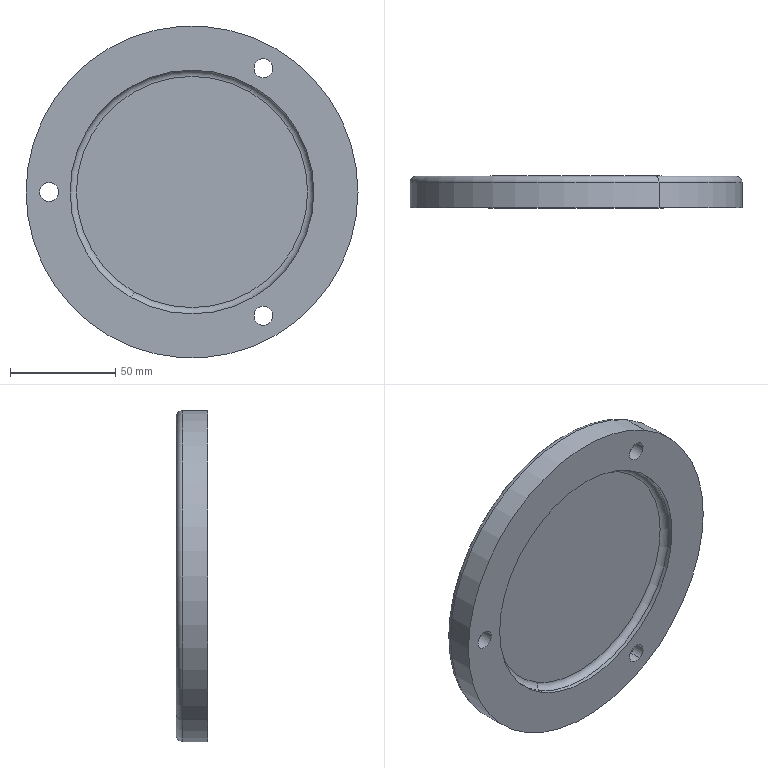Component | SolidWorks | 23-1 | 1 solid | 26 faces | box 158 x 15 x 158 mm | volume 235087 mm3 | cylinder 16 | plane 6 | torus 4 | commonest cylinder face diameters 15 x6 9 x6 116 x2 158 x2
build123d program:
from build123d import *

# Parameters (mm, degrees)
SKETCH1_R           = 79
BOSS_EXTRUDE1_DEPTH = 15
SKETCH2_R           = 58
CUT_EXTRUDE1_DEPTH  = 5
HOLE1_D             = 9
HOLE1_DEPTH         = 99.955
HOLE1_CBORE_D       = 15
HOLE1_CBORE_DEPTH   = 9
CIRPATTERN1_COUNT   = 3
FILLET1_R           = 3
FILLET2_R           = 3


with BuildPart() as part:
    # Sketch1 → Boss-Extrude1 (new body)
    with BuildSketch(Plane(origin=(0, 0, 0), x_dir=(1, 0, 0), z_dir=(0, 1, 0))):
        with Locations(Location((0, 0, 0), (0, 0, 270))):
            Circle(SKETCH1_R)
    extrude(amount=BOSS_EXTRUDE1_DEPTH)

    # Sketch2 → Cut-Extrude1 (cut)
    with BuildSketch(Plane(origin=(0, 15, 0), x_dir=(1, 0, 0), z_dir=(0, 1, 0))):
        with Locations(Location((0, 0, 0), (0, 0, 270))):
            Circle(SKETCH2_R)
    extrude(amount=-CUT_EXTRUDE1_DEPTH, mode=Mode.SUBTRACT)

    # Hole1
    with Locations(Plane(origin=(0, 0, 0), x_dir=(-1, 0, 0), z_dir=(0, -1, 0))):
        with Locations((0, -68)):
            hole1 = CounterBoreHole(HOLE1_D / 2, HOLE1_CBORE_D / 2, HOLE1_CBORE_DEPTH, depth=HOLE1_DEPTH)

    # CirPattern1: Hole1 ×3 about axis
    cirpattern1_axis = Axis((0, 0, 0), (0, 1, 0))
    for i in range(1, CIRPATTERN1_COUNT):
        add(hole1.rotate(cirpattern1_axis, i * 360 / CIRPATTERN1_COUNT), mode=Mode.SUBTRACT)

    # Fillet1
    fillet1_edges = [part.edges().sort_by_distance(p)[0] for p in [
        (0, 10, -58),
    ]]
    fillet(fillet1_edges, radius=FILLET1_R)

    # Fillet2
    fillet2_edges = [part.edges().sort_by_distance(p)[0] for p in [
        (0, 0, -79),
    ]]
    fillet(fillet2_edges, radius=FILLET2_R)


solid = part.part

# Placed as in the assembly
solid = solid.moved(Location((0, 30.2, 0), (180, -90, 0)))
STEP:
#1=COLOUR_RGB('',0.7922,0.8196,0.9333);
#2=FILL_AREA_STYLE_COLOUR('',#1);
#3=FILL_AREA_STYLE('',(#2));
#4=SURFACE_STYLE_FILL_AREA(#3);
#5=SURFACE_SIDE_STYLE('',(#4));
#6=SURFACE_STYLE_USAGE(.BOTH.,#5);
#7=PRESENTATION_STYLE_ASSIGNMENT((#6));
#8=CARTESIAN_POINT('',(-1.496,1.189,-2.591));
#9=VERTEX_POINT('',#8);
#10=CARTESIAN_POINT('',(1.496,1.189,2.591));
#11=VERTEX_POINT('',#10);
#12=CARTESIAN_POINT('',(0.,1.189,-0.));
#13=DIRECTION('',(-0.,1.,0.));
#14=DIRECTION('',(0.5,0.,0.866));
#15=AXIS2_PLACEMENT_3D('',#12,#13,#14);
#16=CIRCLE('',#15,2.992);
#17=EDGE_CURVE('',#9,#11,#16,.T.);
#18=ORIENTED_EDGE('',*,*,#17,.F.);
#19=CARTESIAN_POINT('',(-1.555,1.071,-2.694));
#20=VERTEX_POINT('',#19);
#21=CARTESIAN_POINT('',(-1.496,1.071,-2.591));
#22=DIRECTION('',(-0.866,-0.,0.5));
#23=DIRECTION('',(0.5,0.,0.866));
#24=AXIS2_PLACEMENT_3D('',#21,#22,#23);
#25=CIRCLE('',#24,0.1181);
#26=EDGE_CURVE('',#9,#20,#25,.T.);
#27=ORIENTED_EDGE('',*,*,#26,.T.);
#28=CARTESIAN_POINT('',(1.555,1.071,2.694));
#29=VERTEX_POINT('',#28);
#30=CARTESIAN_POINT('',(0.,1.071,-0.));
#31=DIRECTION('',(0.,-1.,-0.));
#32=DIRECTION('',(0.5,0.,0.866));
#33=AXIS2_PLACEMENT_3D('',#30,#31,#32);
#34=CIRCLE('',#33,3.11);
#35=EDGE_CURVE('',#29,#20,#34,.T.);
#36=ORIENTED_EDGE('',*,*,#35,.F.);
#37=CARTESIAN_POINT('',(1.496,1.071,2.591));
#38=DIRECTION('',(0.866,0.,-0.5));
#39=DIRECTION('',(-0.5,0.,-0.866));
#40=AXIS2_PLACEMENT_3D('',#37,#38,#39);
#41=CIRCLE('',#40,0.1181);
#42=EDGE_CURVE('',#11,#29,#41,.T.);
#43=ORIENTED_EDGE('',*,*,#42,.F.);
#44=EDGE_LOOP('',(#18,#27,#36,#43));
#45=FACE_OUTER_BOUND('',#44,.T.);
#46=CARTESIAN_POINT('',(0.,1.071,-0.));
#47=DIRECTION('',(0.,-1.,-0.));
#48=DIRECTION('',(0.5,0.,0.866));
#49=AXIS2_PLACEMENT_3D('',#46,#47,#48);
#50=TOROIDAL_SURFACE('',#49,2.992,0.1181);
#51=ADVANCED_FACE('',(#45),#50,.T.);
#52=CARTESIAN_POINT('',(-1.083,0.7953,-1.875));
#53=VERTEX_POINT('',#52);
#54=CARTESIAN_POINT('',(1.083,0.7953,1.875));
#55=VERTEX_POINT('',#54);
#56=CARTESIAN_POINT('',(0.,0.7953,-0.));
#57=DIRECTION('',(0.,-1.,-0.));
#58=DIRECTION('',(0.5,0.,0.866));
#59=AXIS2_PLACEMENT_3D('',#56,#57,#58);
#60=CIRCLE('',#59,2.165);
#61=EDGE_CURVE('',#53,#55,#60,.T.);
#62=ORIENTED_EDGE('',*,*,#61,.F.);
#63=CARTESIAN_POINT('',(-1.142,0.6772,-1.978));
#64=VERTEX_POINT('',#63);
#65=CARTESIAN_POINT('',(-1.083,0.6772,-1.875));
#66=DIRECTION('',(-0.866,-0.,0.5));
#67=DIRECTION('',(0.5,0.,0.866));
#68=AXIS2_PLACEMENT_3D('',#65,#66,#67);
#69=CIRCLE('',#68,0.1181);
#70=EDGE_CURVE('',#53,#64,#69,.T.);
#71=ORIENTED_EDGE('',*,*,#70,.T.);
#72=CARTESIAN_POINT('',(1.142,0.6772,1.978));
#73=VERTEX_POINT('',#72);
#74=CARTESIAN_POINT('',(0.,0.6772,-0.));
#75=DIRECTION('',(-0.,1.,0.));
#76=DIRECTION('',(0.5,0.,0.866));
#77=AXIS2_PLACEMENT_3D('',#74,#75,#76);
#78=CIRCLE('',#77,2.283);
#79=EDGE_CURVE('',#73,#64,#78,.T.);
#80=ORIENTED_EDGE('',*,*,#79,.F.);
#81=CARTESIAN_POINT('',(1.083,0.6772,1.875));
#82=DIRECTION('',(0.866,0.,-0.5));
#83=DIRECTION('',(-0.5,0.,-0.866));
#84=AXIS2_PLACEMENT_3D('',#81,#82,#83);
#85=CIRCLE('',#84,0.1181);
#86=EDGE_CURVE('',#55,#73,#85,.T.);
#87=ORIENTED_EDGE('',*,*,#86,.F.);
#88=EDGE_LOOP('',(#62,#71,#80,#87));
#89=FACE_OUTER_BOUND('',#88,.T.);
#90=CARTESIAN_POINT('',(0.,0.6772,-0.));
#91=DIRECTION('',(0.,-1.,-0.));
#92=DIRECTION('',(0.5,0.,0.866));
#93=AXIS2_PLACEMENT_3D('',#90,#91,#92);
#94=TOROIDAL_SURFACE('',#93,2.165,0.1181);
#95=ADVANCED_FACE('',(#89),#94,.F.);
#96=CARTESIAN_POINT('',(-2.972,0.8346,-0.));
#97=VERTEX_POINT('',#96);
#98=CARTESIAN_POINT('',(-2.382,0.8346,-0.));
#99=VERTEX_POINT('',#98);
#100=CARTESIAN_POINT('',(-2.677,0.8346,-0.));
#101=DIRECTION('',(-0.,1.,0.));
#102=DIRECTION('',(1.,0.,0.));
#103=AXIS2_PLACEMENT_3D('',#100,#101,#102);
#104=CIRCLE('',#103,0.2953);
#105=EDGE_CURVE('',#97,#99,#104,.T.);
#106=ORIENTED_EDGE('',*,*,#105,.F.);
#107=CARTESIAN_POINT('',(-2.972,1.189,-0.));
#108=VERTEX_POINT('',#107);
#109=CARTESIAN_POINT('',(-2.972,1.189,-0.));
#110=DIRECTION('',(-0.,1.,0.));
#111=VECTOR('',#110,39.37);
#112=LINE('',#109,#111);
#113=EDGE_CURVE('',#97,#108,#112,.T.);
#114=ORIENTED_EDGE('',*,*,#113,.T.);
#115=CARTESIAN_POINT('',(-2.382,1.189,-0.));
#116=VERTEX_POINT('',#115);
#117=CARTESIAN_POINT('',(-2.677,1.189,-0.));
#118=DIRECTION('',(-0.,1.,0.));
#119=DIRECTION('',(1.,0.,0.));
#120=AXIS2_PLACEMENT_3D('',#117,#118,#119);
#121=CIRCLE('',#120,0.2953);
#122=EDGE_CURVE('',#108,#116,#121,.T.);
#123=ORIENTED_EDGE('',*,*,#122,.T.);
#124=CARTESIAN_POINT('',(-2.382,1.189,-0.));
#125=DIRECTION('',(-0.,1.,0.));
#126=VECTOR('',#125,39.37);
#127=LINE('',#124,#126);
#128=EDGE_CURVE('',#99,#116,#127,.T.);
#129=ORIENTED_EDGE('',*,*,#128,.F.);
#130=EDGE_LOOP('',(#106,#114,#123,#129));
#131=FACE_OUTER_BOUND('',#130,.T.);
#132=CARTESIAN_POINT('',(-2.677,1.189,-0.));
#133=DIRECTION('',(-0.,1.,0.));
#134=DIRECTION('',(1.,0.,0.));
#135=AXIS2_PLACEMENT_3D('',#132,#133,#134);
#136=CYLINDRICAL_SURFACE('',#135,0.2953);
#137=ADVANCED_FACE('',(#131),#136,.F.);
#138=CARTESIAN_POINT('',(-2.5,0.5984,-0.));
#139=VERTEX_POINT('',#138);
#140=CARTESIAN_POINT('',(-2.854,0.5984,-0.));
#141=VERTEX_POINT('',#140);
#142=CARTESIAN_POINT('',(-2.677,0.5984,-0.));
#143=DIRECTION('',(0.,-1.,-0.));
#144=DIRECTION('',(-1.,0.,-0.));
#145=AXIS2_PLACEMENT_3D('',#142,#143,#144);
#146=CIRCLE('',#145,0.1772);
#147=EDGE_CURVE('',#139,#141,#146,.T.);
#148=ORIENTED_EDGE('',*,*,#147,.T.);
#149=CARTESIAN_POINT('',(-2.854,0.8346,-0.));
#150=VERTEX_POINT('',#149);
#151=CARTESIAN_POINT('',(-2.854,1.189,-0.));
#152=DIRECTION('',(-0.,1.,0.));
#153=VECTOR('',#152,39.37);
#154=LINE('',#151,#153);
#155=EDGE_CURVE('',#141,#150,#154,.T.);
#156=ORIENTED_EDGE('',*,*,#155,.T.);
#157=CARTESIAN_POINT('',(-2.5,0.8346,-0.));
#158=VERTEX_POINT('',#157);
#159=CARTESIAN_POINT('',(-2.677,0.8346,-0.));
#160=DIRECTION('',(-0.,1.,0.));
#161=DIRECTION('',(1.,0.,0.));
#162=AXIS2_PLACEMENT_3D('',#159,#160,#161);
#163=CIRCLE('',#162,0.1772);
#164=EDGE_CURVE('',#150,#158,#163,.T.);
#165=ORIENTED_EDGE('',*,*,#164,.T.);
#166=CARTESIAN_POINT('',(-2.5,1.189,-0.));
#167=DIRECTION('',(-0.,1.,0.));
#168=VECTOR('',#167,39.37);
#169=LINE('',#166,#168);
#170=EDGE_CURVE('',#139,#158,#169,.T.);
#171=ORIENTED_EDGE('',*,*,#170,.F.);
#172=EDGE_LOOP('',(#148,#156,#165,#171));
#173=FACE_OUTER_BOUND('',#172,.T.);
#174=CARTESIAN_POINT('',(-2.677,1.189,-0.));
#175=DIRECTION('',(-0.,1.,0.));
#176=DIRECTION('',(1.,0.,0.));
#177=AXIS2_PLACEMENT_3D('',#174,#175,#176);
#178=CYLINDRICAL_SURFACE('',#177,0.1772);
#179=ADVANCED_FACE('',(#173),#178,.F.);
#180=CARTESIAN_POINT('',(1.486,0.8346,-2.574));
#181=VERTEX_POINT('',#180);
#182=CARTESIAN_POINT('',(1.191,0.8346,-2.063));
#183=VERTEX_POINT('',#182);
#184=CARTESIAN_POINT('',(1.339,0.8346,-2.318));
#185=DIRECTION('',(-0.,1.,0.));
#186=DIRECTION('',(-0.5,0.,0.866));
#187=AXIS2_PLACEMENT_3D('',#184,#185,#186);
#188=CIRCLE('',#187,0.2953);
#189=EDGE_CURVE('',#181,#183,#188,.T.);
#190=ORIENTED_EDGE('',*,*,#189,.F.);
#191=CARTESIAN_POINT('',(1.486,1.189,-2.574));
#192=VERTEX_POINT('',#191);
#193=CARTESIAN_POINT('',(1.486,1.189,-2.574));
#194=DIRECTION('',(-0.,1.,0.));
#195=VECTOR('',#194,39.37);
#196=LINE('',#193,#195);
#197=EDGE_CURVE('',#181,#192,#196,.T.);
#198=ORIENTED_EDGE('',*,*,#197,.T.);
#199=CARTESIAN_POINT('',(1.191,1.189,-2.063));
#200=VERTEX_POINT('',#199);
#201=CARTESIAN_POINT('',(1.339,1.189,-2.318));
#202=DIRECTION('',(-0.,1.,0.));
#203=DIRECTION('',(-0.5,0.,0.866));
#204=AXIS2_PLACEMENT_3D('',#201,#202,#203);
#205=CIRCLE('',#204,0.2953);
#206=EDGE_CURVE('',#192,#200,#205,.T.);
#207=ORIENTED_EDGE('',*,*,#206,.T.);
#208=CARTESIAN_POINT('',(1.191,1.189,-2.063));
#209=DIRECTION('',(-0.,1.,0.));
#210=VECTOR('',#209,39.37);
#211=LINE('',#208,#210);
#212=EDGE_CURVE('',#183,#200,#211,.T.);
#213=ORIENTED_EDGE('',*,*,#212,.F.);
#214=EDGE_LOOP('',(#190,#198,#207,#213));
#215=FACE_OUTER_BOUND('',#214,.T.);
#216=CARTESIAN_POINT('',(1.339,1.189,-2.318));
#217=DIRECTION('',(-0.,1.,0.));
#218=DIRECTION('',(-0.5,0.,0.866));
#219=AXIS2_PLACEMENT_3D('',#216,#217,#218);
#220=CYLINDRICAL_SURFACE('',#219,0.2953);
#221=ADVANCED_FACE('',(#215),#220,.F.);
#222=CARTESIAN_POINT('',(1.25,0.5984,-2.165));
#223=VERTEX_POINT('',#222);
#224=CARTESIAN_POINT('',(1.427,0.5984,-2.472));
#225=VERTEX_POINT('',#224);
#226=CARTESIAN_POINT('',(1.339,0.5984,-2.318));
#227=DIRECTION('',(0.,-1.,-0.));
#228=DIRECTION('',(0.5,0.,-0.866));
#229=AXIS2_PLACEMENT_3D('',#226,#227,#228);
#230=CIRCLE('',#229,0.1772);
#231=EDGE_CURVE('',#223,#225,#230,.T.);
#232=ORIENTED_EDGE('',*,*,#231,.T.);
#233=CARTESIAN_POINT('',(1.427,0.8346,-2.472));
#234=VERTEX_POINT('',#233);
#235=CARTESIAN_POINT('',(1.427,1.189,-2.472));
#236=DIRECTION('',(-0.,1.,0.));
#237=VECTOR('',#236,39.37);
#238=LINE('',#235,#237);
#239=EDGE_CURVE('',#225,#234,#238,.T.);
#240=ORIENTED_EDGE('',*,*,#239,.T.);
#241=CARTESIAN_POINT('',(1.25,0.8346,-2.165));
#242=VERTEX_POINT('',#241);
#243=CARTESIAN_POINT('',(1.339,0.8346,-2.318));
#244=DIRECTION('',(-0.,1.,0.));
#245=DIRECTION('',(-0.5,0.,0.866));
#246=AXIS2_PLACEMENT_3D('',#243,#244,#245);
#247=CIRCLE('',#246,0.1772);
#248=EDGE_CURVE('',#234,#242,#247,.T.);
#249=ORIENTED_EDGE('',*,*,#248,.T.);
#250=CARTESIAN_POINT('',(1.25,1.189,-2.165));
#251=DIRECTION('',(-0.,1.,0.));
#252=VECTOR('',#251,39.37);
#253=LINE('',#250,#252);
#254=EDGE_CURVE('',#223,#242,#253,.T.);
#255=ORIENTED_EDGE('',*,*,#254,.F.);
#256=EDGE_LOOP('',(#232,#240,#249,#255));
#257=FACE_OUTER_BOUND('',#256,.T.);
#258=CARTESIAN_POINT('',(1.339,1.189,-2.318));
#259=DIRECTION('',(-0.,1.,0.));
#260=DIRECTION('',(-0.5,0.,0.866));
#261=AXIS2_PLACEMENT_3D('',#258,#259,#260);
#262=CYLINDRICAL_SURFACE('',#261,0.1772);
#263=ADVANCED_FACE('',(#257),#262,.F.);
#264=CARTESIAN_POINT('',(1.486,0.8346,2.574));
#265=VERTEX_POINT('',#264);
#266=CARTESIAN_POINT('',(1.191,0.8346,2.063));
#267=VERTEX_POINT('',#266);
#268=CARTESIAN_POINT('',(1.339,0.8346,2.318));
#269=DIRECTION('',(-0.,1.,0.));
#270=DIRECTION('',(-0.5,0.,-0.866));
#271=AXIS2_PLACEMENT_3D('',#268,#269,#270);
#272=CIRCLE('',#271,0.2953);
#273=EDGE_CURVE('',#265,#267,#272,.T.);
#274=ORIENTED_EDGE('',*,*,#273,.F.);
#275=CARTESIAN_POINT('',(1.486,1.189,2.574));
#276=VERTEX_POINT('',#275);
#277=CARTESIAN_POINT('',(1.486,1.189,2.574));
#278=DIRECTION('',(-0.,1.,0.));
#279=VECTOR('',#278,39.37);
#280=LINE('',#277,#279);
#281=EDGE_CURVE('',#265,#276,#280,.T.);
#282=ORIENTED_EDGE('',*,*,#281,.T.);
#283=CARTESIAN_POINT('',(1.191,1.189,2.063));
#284=VERTEX_POINT('',#283);
#285=CARTESIAN_POINT('',(1.339,1.189,2.318));
#286=DIRECTION('',(-0.,1.,0.));
#287=DIRECTION('',(-0.5,0.,-0.866));
#288=AXIS2_PLACEMENT_3D('',#285,#286,#287);
#289=CIRCLE('',#288,0.2953);
#290=EDGE_CURVE('',#276,#284,#289,.T.);
#291=ORIENTED_EDGE('',*,*,#290,.T.);
#292=CARTESIAN_POINT('',(1.191,1.189,2.063));
#293=DIRECTION('',(-0.,1.,0.));
#294=VECTOR('',#293,39.37);
#295=LINE('',#292,#294);
#296=EDGE_CURVE('',#267,#284,#295,.T.);
#297=ORIENTED_EDGE('',*,*,#296,.F.);
#298=EDGE_LOOP('',(#274,#282,#291,#297));
#299=FACE_OUTER_BOUND('',#298,.T.);
#300=CARTESIAN_POINT('',(1.339,1.189,2.318));
#301=DIRECTION('',(-0.,1.,0.));
#302=DIRECTION('',(-0.5,0.,-0.866));
#303=AXIS2_PLACEMENT_3D('',#300,#301,#302);
#304=CYLINDRICAL_SURFACE('',#303,0.2953);
#305=ADVANCED_FACE('',(#299),#304,.F.);
#306=CARTESIAN_POINT('',(1.25,0.5984,2.165));
#307=VERTEX_POINT('',#306);
#308=CARTESIAN_POINT('',(1.427,0.5984,2.472));
#309=VERTEX_POINT('',#308);
#310=CARTESIAN_POINT('',(1.339,0.5984,2.318));
#311=DIRECTION('',(0.,-1.,-0.));
#312=DIRECTION('',(0.5,0.,0.866));
#313=AXIS2_PLACEMENT_3D('',#310,#311,#312);
#314=CIRCLE('',#313,0.1772);
#315=EDGE_CURVE('',#307,#309,#314,.T.);
#316=ORIENTED_EDGE('',*,*,#315,.T.);
#317=CARTESIAN_POINT('',(1.427,0.8346,2.472));
#318=VERTEX_POINT('',#317);
#319=CARTESIAN_POINT('',(1.427,1.189,2.472));
#320=DIRECTION('',(-0.,1.,0.));
#321=VECTOR('',#320,39.37);
#322=LINE('',#319,#321);
#323=EDGE_CURVE('',#309,#318,#322,.T.);
#324=ORIENTED_EDGE('',*,*,#323,.T.);
#325=CARTESIAN_POINT('',(1.25,0.8346,2.165));
#326=VERTEX_POINT('',#325);
#327=CARTESIAN_POINT('',(1.339,0.8346,2.318));
#328=DIRECTION('',(-0.,1.,0.));
#329=DIRECTION('',(-0.5,0.,-0.866));
#330=AXIS2_PLACEMENT_3D('',#327,#328,#329);
#331=CIRCLE('',#330,0.1772);
#332=EDGE_CURVE('',#318,#326,#331,.T.);
#333=ORIENTED_EDGE('',*,*,#332,.T.);
#334=CARTESIAN_POINT('',(1.25,1.189,2.165));
#335=DIRECTION('',(-0.,1.,0.));
#336=VECTOR('',#335,39.37);
#337=LINE('',#334,#336);
#338=EDGE_CURVE('',#307,#326,#337,.T.);
#339=ORIENTED_EDGE('',*,*,#338,.F.);
#340=EDGE_LOOP('',(#316,#324,#333,#339));
#341=FACE_OUTER_BOUND('',#340,.T.);
#342=CARTESIAN_POINT('',(1.339,1.189,2.318));
#343=DIRECTION('',(-0.,1.,0.));
#344=DIRECTION('',(-0.5,0.,-0.866));
#345=AXIS2_PLACEMENT_3D('',#342,#343,#344);
#346=CYLINDRICAL_SURFACE('',#345,0.1772);
#347=ADVANCED_FACE('',(#341),#346,.F.);
#348=ORIENTED_EDGE('',*,*,#79,.T.);
#349=CARTESIAN_POINT('',(-1.142,0.5984,-1.978));
#350=VERTEX_POINT('',#349);
#351=CARTESIAN_POINT('',(-1.142,0.7953,-1.978));
#352=DIRECTION('',(0.,-1.,-0.));
#353=VECTOR('',#352,39.37);
#354=LINE('',#351,#353);
#355=EDGE_CURVE('',#64,#350,#354,.T.);
#356=ORIENTED_EDGE('',*,*,#355,.T.);
#357=CARTESIAN_POINT('',(1.142,0.5984,1.978));
#358=VERTEX_POINT('',#357);
#359=CARTESIAN_POINT('',(0.,0.5984,-0.));
#360=DIRECTION('',(0.,-1.,-0.));
#361=DIRECTION('',(0.5,0.,0.866));
#362=AXIS2_PLACEMENT_3D('',#359,#360,#361);
#363=CIRCLE('',#362,2.283);
#364=EDGE_CURVE('',#350,#358,#363,.T.);
#365=ORIENTED_EDGE('',*,*,#364,.T.);
#366=CARTESIAN_POINT('',(1.142,0.7953,1.978));
#367=DIRECTION('',(0.,-1.,-0.));
#368=VECTOR('',#367,39.37);
#369=LINE('',#366,#368);
#370=EDGE_CURVE('',#73,#358,#369,.T.);
#371=ORIENTED_EDGE('',*,*,#370,.F.);
#372=EDGE_LOOP('',(#348,#356,#365,#371));
#373=FACE_OUTER_BOUND('',#372,.T.);
#374=CARTESIAN_POINT('',(0.,0.7953,-0.));
#375=DIRECTION('',(0.,-1.,-0.));
#376=DIRECTION('',(0.5,0.,0.866));
#377=AXIS2_PLACEMENT_3D('',#374,#375,#376);
#378=CYLINDRICAL_SURFACE('',#377,2.283);
#379=ADVANCED_FACE('',(#373),#378,.F.);
#380=CARTESIAN_POINT('',(1.555,0.5984,2.694));
#381=VERTEX_POINT('',#380);
#382=CARTESIAN_POINT('',(-1.555,0.5984,-2.694));
#383=VERTEX_POINT('',#382);
#384=CARTESIAN_POINT('',(0.,0.5984,-0.));
#385=DIRECTION('',(0.,-1.,-0.));
#386=DIRECTION('',(0.5,0.,0.866));
#387=AXIS2_PLACEMENT_3D('',#384,#385,#386);
#388=CIRCLE('',#387,3.11);
#389=EDGE_CURVE('',#381,#383,#388,.T.);
#390=ORIENTED_EDGE('',*,*,#389,.F.);
#391=CARTESIAN_POINT('',(1.555,0.5984,2.694));
#392=DIRECTION('',(-0.,1.,0.));
#393=VECTOR('',#392,39.37);
#394=LINE('',#391,#393);
#395=EDGE_CURVE('',#381,#29,#394,.T.);
#396=ORIENTED_EDGE('',*,*,#395,.T.);
#397=ORIENTED_EDGE('',*,*,#35,.T.);
#398=CARTESIAN_POINT('',(-1.555,0.5984,-2.694));
#399=DIRECTION('',(-0.,1.,0.));
#400=VECTOR('',#399,39.37);
#401=LINE('',#398,#400);
#402=EDGE_CURVE('',#383,#20,#401,.T.);
#403=ORIENTED_EDGE('',*,*,#402,.F.);
#404=EDGE_LOOP('',(#390,#396,#397,#403));
#405=FACE_OUTER_BOUND('',#404,.T.);
#406=CARTESIAN_POINT('',(0.,0.5984,-0.));
#407=DIRECTION('',(-0.,1.,0.));
#408=DIRECTION('',(-0.5,-0.,-0.866));
#409=AXIS2_PLACEMENT_3D('',#406,#407,#408);
#410=CYLINDRICAL_SURFACE('',#409,3.11);
#411=ADVANCED_FACE('',(#405),#410,.T.);
#412=ORIENTED_EDGE('',*,*,#395,.F.);
#413=CARTESIAN_POINT('',(0.,0.5984,-0.));
#414=DIRECTION('',(0.,-1.,-0.));
#415=DIRECTION('',(0.5,0.,0.866));
#416=AXIS2_PLACEMENT_3D('',#413,#414,#415);
#417=CIRCLE('',#416,3.11);
#418=EDGE_CURVE('',#383,#381,#417,.T.);
#419=ORIENTED_EDGE('',*,*,#418,.F.);
#420=ORIENTED_EDGE('',*,*,#402,.T.);
#421=CARTESIAN_POINT('',(0.,1.071,-0.));
#422=DIRECTION('',(0.,-1.,-0.));
#423=DIRECTION('',(0.5,0.,0.866));
#424=AXIS2_PLACEMENT_3D('',#421,#422,#423);
#425=CIRCLE('',#424,3.11);
#426=EDGE_CURVE('',#20,#29,#425,.T.);
#427=ORIENTED_EDGE('',*,*,#426,.T.);
#428=EDGE_LOOP('',(#412,#419,#420,#427));
#429=FACE_OUTER_BOUND('',#428,.T.);
#430=CARTESIAN_POINT('',(0.,0.5984,-0.));
#431=DIRECTION('',(-0.,1.,0.));
#432=DIRECTION('',(-0.5,-0.,-0.866));
#433=AXIS2_PLACEMENT_3D('',#430,#431,#432);
#434=CYLINDRICAL_SURFACE('',#433,3.11);
#435=ADVANCED_FACE('',(#429),#434,.T.);
#436=ORIENTED_EDGE('',*,*,#147,.F.);
#437=CARTESIAN_POINT('',(-2.677,0.5984,-0.));
#438=DIRECTION('',(0.,-1.,-0.));
#439=DIRECTION('',(-1.,0.,-0.));
#440=AXIS2_PLACEMENT_3D('',#437,#438,#439);
#441=CIRCLE('',#440,0.1772);
#442=EDGE_CURVE('',#141,#139,#441,.T.);
#443=ORIENTED_EDGE('',*,*,#442,.F.);
#444=EDGE_LOOP('',(#436,#443));
#445=FACE_BOUND('',#444,.T.);
#446=ORIENTED_EDGE('',*,*,#231,.F.);
#447=CARTESIAN_POINT('',(1.339,0.5984,-2.318));
#448=DIRECTION('',(0.,-1.,-0.));
#449=DIRECTION('',(0.5,0.,-0.866));
#450=AXIS2_PLACEMENT_3D('',#447,#448,#449);
#451=CIRCLE('',#450,0.1772);
#452=EDGE_CURVE('',#225,#223,#451,.T.);
#453=ORIENTED_EDGE('',*,*,#452,.F.);
#454=EDGE_LOOP('',(#446,#453));
#455=FACE_BOUND('',#454,.T.);
#456=ORIENTED_EDGE('',*,*,#315,.F.);
#457=CARTESIAN_POINT('',(1.339,0.5984,2.318));
#458=DIRECTION('',(0.,-1.,-0.));
#459=DIRECTION('',(0.5,0.,0.866));
#460=AXIS2_PLACEMENT_3D('',#457,#458,#459);
#461=CIRCLE('',#460,0.1772);
#462=EDGE_CURVE('',#309,#307,#461,.T.);
#463=ORIENTED_EDGE('',*,*,#462,.F.);
#464=EDGE_LOOP('',(#456,#463));
#465=FACE_BOUND('',#464,.T.);
#466=CARTESIAN_POINT('',(0.,0.5984,-0.));
#467=DIRECTION('',(0.,-1.,-0.));
#468=DIRECTION('',(0.5,0.,0.866));
#469=AXIS2_PLACEMENT_3D('',#466,#467,#468);
#470=CIRCLE('',#469,2.283);
#471=EDGE_CURVE('',#358,#350,#470,.T.);
#472=ORIENTED_EDGE('',*,*,#471,.F.);
#473=ORIENTED_EDGE('',*,*,#364,.F.);
#474=EDGE_LOOP('',(#472,#473));
#475=FACE_BOUND('',#474,.T.);
#476=ORIENTED_EDGE('',*,*,#418,.T.);
#477=ORIENTED_EDGE('',*,*,#389,.T.);
#478=EDGE_LOOP('',(#476,#477));
#479=FACE_OUTER_BOUND('',#478,.T.);
#480=CARTESIAN_POINT('',(0.,0.5984,-0.));
#481=DIRECTION('',(0.,-1.,-0.));
#482=DIRECTION('',(0.5,0.,0.866));
#483=AXIS2_PLACEMENT_3D('',#480,#481,#482);
#484=PLANE('',#483);
#485=ADVANCED_FACE('',(#445,#455,#465,#475,#479),#484,.T.);
#486=CARTESIAN_POINT('',(0.,1.189,-0.));
#487=DIRECTION('',(-0.,1.,0.));
#488=DIRECTION('',(0.5,0.,0.866));
#489=AXIS2_PLACEMENT_3D('',#486,#487,#488);
#490=CIRCLE('',#489,2.992);
#491=EDGE_CURVE('',#11,#9,#490,.T.);
#492=ORIENTED_EDGE('',*,*,#491,.T.);
#493=ORIENTED_EDGE('',*,*,#17,.T.);
#494=EDGE_LOOP('',(#492,#493));
#495=FACE_OUTER_BOUND('',#494,.T.);
#496=CARTESIAN_POINT('',(-2.677,1.189,-0.));
#497=DIRECTION('',(-0.,1.,0.));
#498=DIRECTION('',(1.,0.,0.));
#499=AXIS2_PLACEMENT_3D('',#496,#497,#498);
#500=CIRCLE('',#499,0.2953);
#501=EDGE_CURVE('',#116,#108,#500,.T.);
#502=ORIENTED_EDGE('',*,*,#501,.F.);
#503=ORIENTED_EDGE('',*,*,#122,.F.);
#504=EDGE_LOOP('',(#502,#503));
#505=FACE_BOUND('',#504,.T.);
#506=CARTESIAN_POINT('',(1.339,1.189,-2.318));
#507=DIRECTION('',(-0.,1.,0.));
#508=DIRECTION('',(-0.5,0.,0.866));
#509=AXIS2_PLACEMENT_3D('',#506,#507,#508);
#510=CIRCLE('',#509,0.2953);
#511=EDGE_CURVE('',#200,#192,#510,.T.);
#512=ORIENTED_EDGE('',*,*,#511,.F.);
#513=ORIENTED_EDGE('',*,*,#206,.F.);
#514=EDGE_LOOP('',(#512,#513));
#515=FACE_BOUND('',#514,.T.);
#516=CARTESIAN_POINT('',(1.339,1.189,2.318));
#517=DIRECTION('',(-0.,1.,0.));
#518=DIRECTION('',(-0.5,0.,-0.866));
#519=AXIS2_PLACEMENT_3D('',#516,#517,#518);
#520=CIRCLE('',#519,0.2953);
#521=EDGE_CURVE('',#284,#276,#520,.T.);
#522=ORIENTED_EDGE('',*,*,#521,.F.);
#523=ORIENTED_EDGE('',*,*,#290,.F.);
#524=EDGE_LOOP('',(#522,#523));
#525=FACE_BOUND('',#524,.T.);
#526=CARTESIAN_POINT('',(0.,1.189,-0.));
#527=DIRECTION('',(0.,-1.,-0.));
#528=DIRECTION('',(0.5,0.,0.866));
#529=AXIS2_PLACEMENT_3D('',#526,#527,#528);
#530=PLANE('',#529);
#531=ADVANCED_FACE('',(#495,#505,#515,#525),#530,.F.);
#532=ORIENTED_EDGE('',*,*,#355,.F.);
#533=CARTESIAN_POINT('',(0.,0.6772,-0.));
#534=DIRECTION('',(-0.,1.,0.));
#535=DIRECTION('',(0.5,0.,0.866));
#536=AXIS2_PLACEMENT_3D('',#533,#534,#535);
#537=CIRCLE('',#536,2.283);
#538=EDGE_CURVE('',#64,#73,#537,.T.);
#539=ORIENTED_EDGE('',*,*,#538,.T.);
#540=ORIENTED_EDGE('',*,*,#370,.T.);
#541=ORIENTED_EDGE('',*,*,#471,.T.);
#542=EDGE_LOOP('',(#532,#539,#540,#541));
#543=FACE_OUTER_BOUND('',#542,.T.);
#544=CARTESIAN_POINT('',(0.,0.7953,-0.));
#545=DIRECTION('',(0.,-1.,-0.));
#546=DIRECTION('',(0.5,0.,0.866));
#547=AXIS2_PLACEMENT_3D('',#544,#545,#546);
#548=CYLINDRICAL_SURFACE('',#547,2.283);
#549=ADVANCED_FACE('',(#543),#548,.F.);
#550=CARTESIAN_POINT('',(0.,0.7953,-0.));
#551=DIRECTION('',(0.,-1.,-0.));
#552=DIRECTION('',(0.5,0.,0.866));
#553=AXIS2_PLACEMENT_3D('',#550,#551,#552);
#554=CIRCLE('',#553,2.165);
#555=EDGE_CURVE('',#55,#53,#554,.T.);
#556=ORIENTED_EDGE('',*,*,#555,.T.);
#557=ORIENTED_EDGE('',*,*,#61,.T.);
#558=EDGE_LOOP('',(#556,#557));
#559=FACE_OUTER_BOUND('',#558,.T.);
#560=CARTESIAN_POINT('',(0.,0.7953,-0.));
#561=DIRECTION('',(0.,-1.,-0.));
#562=DIRECTION('',(0.5,0.,0.866));
#563=AXIS2_PLACEMENT_3D('',#560,#561,#562);
#564=PLANE('',#563);
#565=ADVANCED_FACE('',(#559),#564,.T.);
#566=ORIENTED_EDGE('',*,*,#323,.F.);
#567=ORIENTED_EDGE('',*,*,#462,.T.);
#568=ORIENTED_EDGE('',*,*,#338,.T.);
#569=CARTESIAN_POINT('',(1.339,0.8346,2.318));
#570=DIRECTION('',(-0.,1.,0.));
#571=DIRECTION('',(-0.5,0.,-0.866));
#572=AXIS2_PLACEMENT_3D('',#569,#570,#571);
#573=CIRCLE('',#572,0.1772);
#574=EDGE_CURVE('',#326,#318,#573,.T.);
#575=ORIENTED_EDGE('',*,*,#574,.T.);
#576=EDGE_LOOP('',(#566,#567,#568,#575));
#577=FACE_OUTER_BOUND('',#576,.T.);
#578=CARTESIAN_POINT('',(1.339,1.189,2.318));
#579=DIRECTION('',(-0.,1.,0.));
#580=DIRECTION('',(-0.5,0.,-0.866));
#581=AXIS2_PLACEMENT_3D('',#578,#579,#580);
#582=CYLINDRICAL_SURFACE('',#581,0.1772);
#583=ADVANCED_FACE('',(#577),#582,.F.);
#584=ORIENTED_EDGE('',*,*,#574,.F.);
#585=ORIENTED_EDGE('',*,*,#332,.F.);
#586=EDGE_LOOP('',(#584,#585));
#587=FACE_BOUND('',#586,.T.);
#588=CARTESIAN_POINT('',(1.339,0.8346,2.318));
#589=DIRECTION('',(-0.,1.,0.));
#590=DIRECTION('',(-0.5,0.,-0.866));
#591=AXIS2_PLACEMENT_3D('',#588,#589,#590);
#592=CIRCLE('',#591,0.2953);
#593=EDGE_CURVE('',#267,#265,#592,.T.);
#594=ORIENTED_EDGE('',*,*,#593,.T.);
#595=ORIENTED_EDGE('',*,*,#273,.T.);
#596=EDGE_LOOP('',(#594,#595));
#597=FACE_OUTER_BOUND('',#596,.T.);
#598=CARTESIAN_POINT('',(1.185,0.8346,2.407));
#599=DIRECTION('',(0.,-1.,-0.));
#600=DIRECTION('',(0.5,0.,0.866));
#601=AXIS2_PLACEMENT_3D('',#598,#599,#600);
#602=PLANE('',#601);
#603=ADVANCED_FACE('',(#587,#597),#602,.F.);
#604=ORIENTED_EDGE('',*,*,#281,.F.);
#605=ORIENTED_EDGE('',*,*,#593,.F.);
#606=ORIENTED_EDGE('',*,*,#296,.T.);
#607=ORIENTED_EDGE('',*,*,#521,.T.);
#608=EDGE_LOOP('',(#604,#605,#606,#607));
#609=FACE_OUTER_BOUND('',#608,.T.);
#610=CARTESIAN_POINT('',(1.339,1.189,2.318));
#611=DIRECTION('',(-0.,1.,0.));
#612=DIRECTION('',(-0.5,0.,-0.866));
#613=AXIS2_PLACEMENT_3D('',#610,#611,#612);
#614=CYLINDRICAL_SURFACE('',#613,0.2953);
#615=ADVANCED_FACE('',(#609),#614,.F.);
#616=ORIENTED_EDGE('',*,*,#239,.F.);
#617=ORIENTED_EDGE('',*,*,#452,.T.);
#618=ORIENTED_EDGE('',*,*,#254,.T.);
#619=CARTESIAN_POINT('',(1.339,0.8346,-2.318));
#620=DIRECTION('',(-0.,1.,0.));
#621=DIRECTION('',(-0.5,0.,0.866));
#622=AXIS2_PLACEMENT_3D('',#619,#620,#621);
#623=CIRCLE('',#622,0.1772);
#624=EDGE_CURVE('',#242,#234,#623,.T.);
#625=ORIENTED_EDGE('',*,*,#624,.T.);
#626=EDGE_LOOP('',(#616,#617,#618,#625));
#627=FACE_OUTER_BOUND('',#626,.T.);
#628=CARTESIAN_POINT('',(1.339,1.189,-2.318));
#629=DIRECTION('',(-0.,1.,0.));
#630=DIRECTION('',(-0.5,0.,0.866));
#631=AXIS2_PLACEMENT_3D('',#628,#629,#630);
#632=CYLINDRICAL_SURFACE('',#631,0.1772);
#633=ADVANCED_FACE('',(#627),#632,.F.);
#634=ORIENTED_EDGE('',*,*,#624,.F.);
#635=ORIENTED_EDGE('',*,*,#248,.F.);
#636=EDGE_LOOP('',(#634,#635));
#637=FACE_BOUND('',#636,.T.);
#638=CARTESIAN_POINT('',(1.339,0.8346,-2.318));
#639=DIRECTION('',(-0.,1.,0.));
#640=DIRECTION('',(-0.5,0.,0.866));
#641=AXIS2_PLACEMENT_3D('',#638,#639,#640);
#642=CIRCLE('',#641,0.2953);
#643=EDGE_CURVE('',#183,#181,#642,.T.);
#644=ORIENTED_EDGE('',*,*,#643,.T.);
#645=ORIENTED_EDGE('',*,*,#189,.T.);
#646=EDGE_LOOP('',(#644,#645));
#647=FACE_OUTER_BOUND('',#646,.T.);
#648=CARTESIAN_POINT('',(1.492,0.8346,-2.23));
#649=DIRECTION('',(0.,-1.,-0.));
#650=DIRECTION('',(0.5,0.,-0.866));
#651=AXIS2_PLACEMENT_3D('',#648,#649,#650);
#652=PLANE('',#651);
#653=ADVANCED_FACE('',(#637,#647),#652,.F.);
#654=ORIENTED_EDGE('',*,*,#197,.F.);
#655=ORIENTED_EDGE('',*,*,#643,.F.);
#656=ORIENTED_EDGE('',*,*,#212,.T.);
#657=ORIENTED_EDGE('',*,*,#511,.T.);
#658=EDGE_LOOP('',(#654,#655,#656,#657));
#659=FACE_OUTER_BOUND('',#658,.T.);
#660=CARTESIAN_POINT('',(1.339,1.189,-2.318));
#661=DIRECTION('',(-0.,1.,0.));
#662=DIRECTION('',(-0.5,0.,0.866));
#663=AXIS2_PLACEMENT_3D('',#660,#661,#662);
#664=CYLINDRICAL_SURFACE('',#663,0.2953);
#665=ADVANCED_FACE('',(#659),#664,.F.);
#666=ORIENTED_EDGE('',*,*,#155,.F.);
#667=ORIENTED_EDGE('',*,*,#442,.T.);
#668=ORIENTED_EDGE('',*,*,#170,.T.);
#669=CARTESIAN_POINT('',(-2.677,0.8346,-0.));
#670=DIRECTION('',(-0.,1.,0.));
#671=DIRECTION('',(1.,0.,0.));
#672=AXIS2_PLACEMENT_3D('',#669,#670,#671);
#673=CIRCLE('',#672,0.1772);
#674=EDGE_CURVE('',#158,#150,#673,.T.);
#675=ORIENTED_EDGE('',*,*,#674,.T.);
#676=EDGE_LOOP('',(#666,#667,#668,#675));
#677=FACE_OUTER_BOUND('',#676,.T.);
#678=CARTESIAN_POINT('',(-2.677,1.189,-0.));
#679=DIRECTION('',(-0.,1.,0.));
#680=DIRECTION('',(1.,0.,0.));
#681=AXIS2_PLACEMENT_3D('',#678,#679,#680);
#682=CYLINDRICAL_SURFACE('',#681,0.1772);
#683=ADVANCED_FACE('',(#677),#682,.F.);
#684=ORIENTED_EDGE('',*,*,#674,.F.);
#685=ORIENTED_EDGE('',*,*,#164,.F.);
#686=EDGE_LOOP('',(#684,#685));
#687=FACE_BOUND('',#686,.T.);
#688=CARTESIAN_POINT('',(-2.677,0.8346,-0.));
#689=DIRECTION('',(-0.,1.,0.));
#690=DIRECTION('',(1.,0.,0.));
#691=AXIS2_PLACEMENT_3D('',#688,#689,#690);
#692=CIRCLE('',#691,0.2953);
#693=EDGE_CURVE('',#99,#97,#692,.T.);
#694=ORIENTED_EDGE('',*,*,#693,.T.);
#695=ORIENTED_EDGE('',*,*,#105,.T.);
#696=EDGE_LOOP('',(#694,#695));
#697=FACE_OUTER_BOUND('',#696,.T.);
#698=CARTESIAN_POINT('',(-2.677,0.8346,-0.1772));
#699=DIRECTION('',(0.,-1.,-0.));
#700=DIRECTION('',(-1.,-0.,-0.));
#701=AXIS2_PLACEMENT_3D('',#698,#699,#700);
#702=PLANE('',#701);
#703=ADVANCED_FACE('',(#687,#697),#702,.F.);
#704=ORIENTED_EDGE('',*,*,#113,.F.);
#705=ORIENTED_EDGE('',*,*,#693,.F.);
#706=ORIENTED_EDGE('',*,*,#128,.T.);
#707=ORIENTED_EDGE('',*,*,#501,.T.);
#708=EDGE_LOOP('',(#704,#705,#706,#707));
#709=FACE_OUTER_BOUND('',#708,.T.);
#710=CARTESIAN_POINT('',(-2.677,1.189,-0.));
#711=DIRECTION('',(-0.,1.,0.));
#712=DIRECTION('',(1.,0.,0.));
#713=AXIS2_PLACEMENT_3D('',#710,#711,#712);
#714=CYLINDRICAL_SURFACE('',#713,0.2953);
#715=ADVANCED_FACE('',(#709),#714,.F.);
#716=ORIENTED_EDGE('',*,*,#70,.F.);
#717=ORIENTED_EDGE('',*,*,#555,.F.);
#718=ORIENTED_EDGE('',*,*,#86,.T.);
#719=ORIENTED_EDGE('',*,*,#538,.F.);
#720=EDGE_LOOP('',(#716,#717,#718,#719));
#721=FACE_OUTER_BOUND('',#720,.T.);
#722=CARTESIAN_POINT('',(0.,0.6772,-0.));
#723=DIRECTION('',(0.,-1.,-0.));
#724=DIRECTION('',(0.5,0.,0.866));
#725=AXIS2_PLACEMENT_3D('',#722,#723,#724);
#726=TOROIDAL_SURFACE('',#725,2.165,0.1181);
#727=ADVANCED_FACE('',(#721),#726,.F.);
#728=ORIENTED_EDGE('',*,*,#26,.F.);
#729=ORIENTED_EDGE('',*,*,#491,.F.);
#730=ORIENTED_EDGE('',*,*,#42,.T.);
#731=ORIENTED_EDGE('',*,*,#426,.F.);
#732=EDGE_LOOP('',(#728,#729,#730,#731));
#733=FACE_OUTER_BOUND('',#732,.T.);
#734=CARTESIAN_POINT('',(0.,1.071,-0.));
#735=DIRECTION('',(0.,-1.,-0.));
#736=DIRECTION('',(0.5,0.,0.866));
#737=AXIS2_PLACEMENT_3D('',#734,#735,#736);
#738=TOROIDAL_SURFACE('',#737,2.992,0.1181);
#739=ADVANCED_FACE('',(#733),#738,.T.);
#740=CLOSED_SHELL('',(#51,#95,#137,#179,#221,#263,#305,#347,#379,#411,#435,#485,#531,#549,#565,#583,#603,#615,#633,#653,#665,#683,#703,#715,#727,#739));
#741=MANIFOLD_SOLID_BREP('',#740);
#742=STYLED_ITEM('',(#7),#741);
#743=PRESENTATION_LAYER_ASSIGNMENT('','',(#742));
#744=(LENGTH_UNIT()NAMED_UNIT(*)SI_UNIT($,.METRE.));
#745=LENGTH_MEASURE_WITH_UNIT(LENGTH_MEASURE(0.0254),#744);
#746=DIMENSIONAL_EXPONENTS(1.,0.,0.,0.,0.,0.,0.);
#747=(CONVERSION_BASED_UNIT('',#745)LENGTH_UNIT()NAMED_UNIT(#746));
#748=UNCERTAINTY_MEASURE_WITH_UNIT(LENGTH_MEASURE(0.00001),#747,'','');
#749=(NAMED_UNIT(*)PLANE_ANGLE_UNIT()SI_UNIT($,.RADIAN.));
#750=(NAMED_UNIT(*)SI_UNIT($,.STERADIAN.)SOLID_ANGLE_UNIT());
#751=(GEOMETRIC_REPRESENTATION_CONTEXT(3)GLOBAL_UNCERTAINTY_ASSIGNED_CONTEXT((#748))GLOBAL_UNIT_ASSIGNED_CONTEXT((#747,#749,#750))REPRESENTATION_CONTEXT('',''));
#752=MECHANICAL_DESIGN_GEOMETRIC_PRESENTATION_REPRESENTATION('',(#742),#751);
#753=CARTESIAN_POINT('',(0.,0.,0.));
#754=DIRECTION('',(0.,0.,1.));
#755=DIRECTION('',(1.,0.,0.));
#756=AXIS2_PLACEMENT_3D('',#753,#754,#755);
#757=(LENGTH_UNIT()NAMED_UNIT(*)SI_UNIT($,.METRE.));
#758=LENGTH_MEASURE_WITH_UNIT(LENGTH_MEASURE(0.0254),#757);
#759=DIMENSIONAL_EXPONENTS(1.,0.,0.,0.,0.,0.,0.);
#760=(CONVERSION_BASED_UNIT('',#758)LENGTH_UNIT()NAMED_UNIT(#759));
#761=UNCERTAINTY_MEASURE_WITH_UNIT(LENGTH_MEASURE(0.00001),#760,'','');
#762=(NAMED_UNIT(*)PLANE_ANGLE_UNIT()SI_UNIT($,.RADIAN.));
#763=(NAMED_UNIT(*)SI_UNIT($,.STERADIAN.)SOLID_ANGLE_UNIT());
#764=(GEOMETRIC_REPRESENTATION_CONTEXT(3)GLOBAL_UNCERTAINTY_ASSIGNED_CONTEXT((#761))GLOBAL_UNIT_ASSIGNED_CONTEXT((#760,#762,#763))REPRESENTATION_CONTEXT('',''));
#765=ADVANCED_BREP_SHAPE_REPRESENTATION('',(#741,#756),#764);